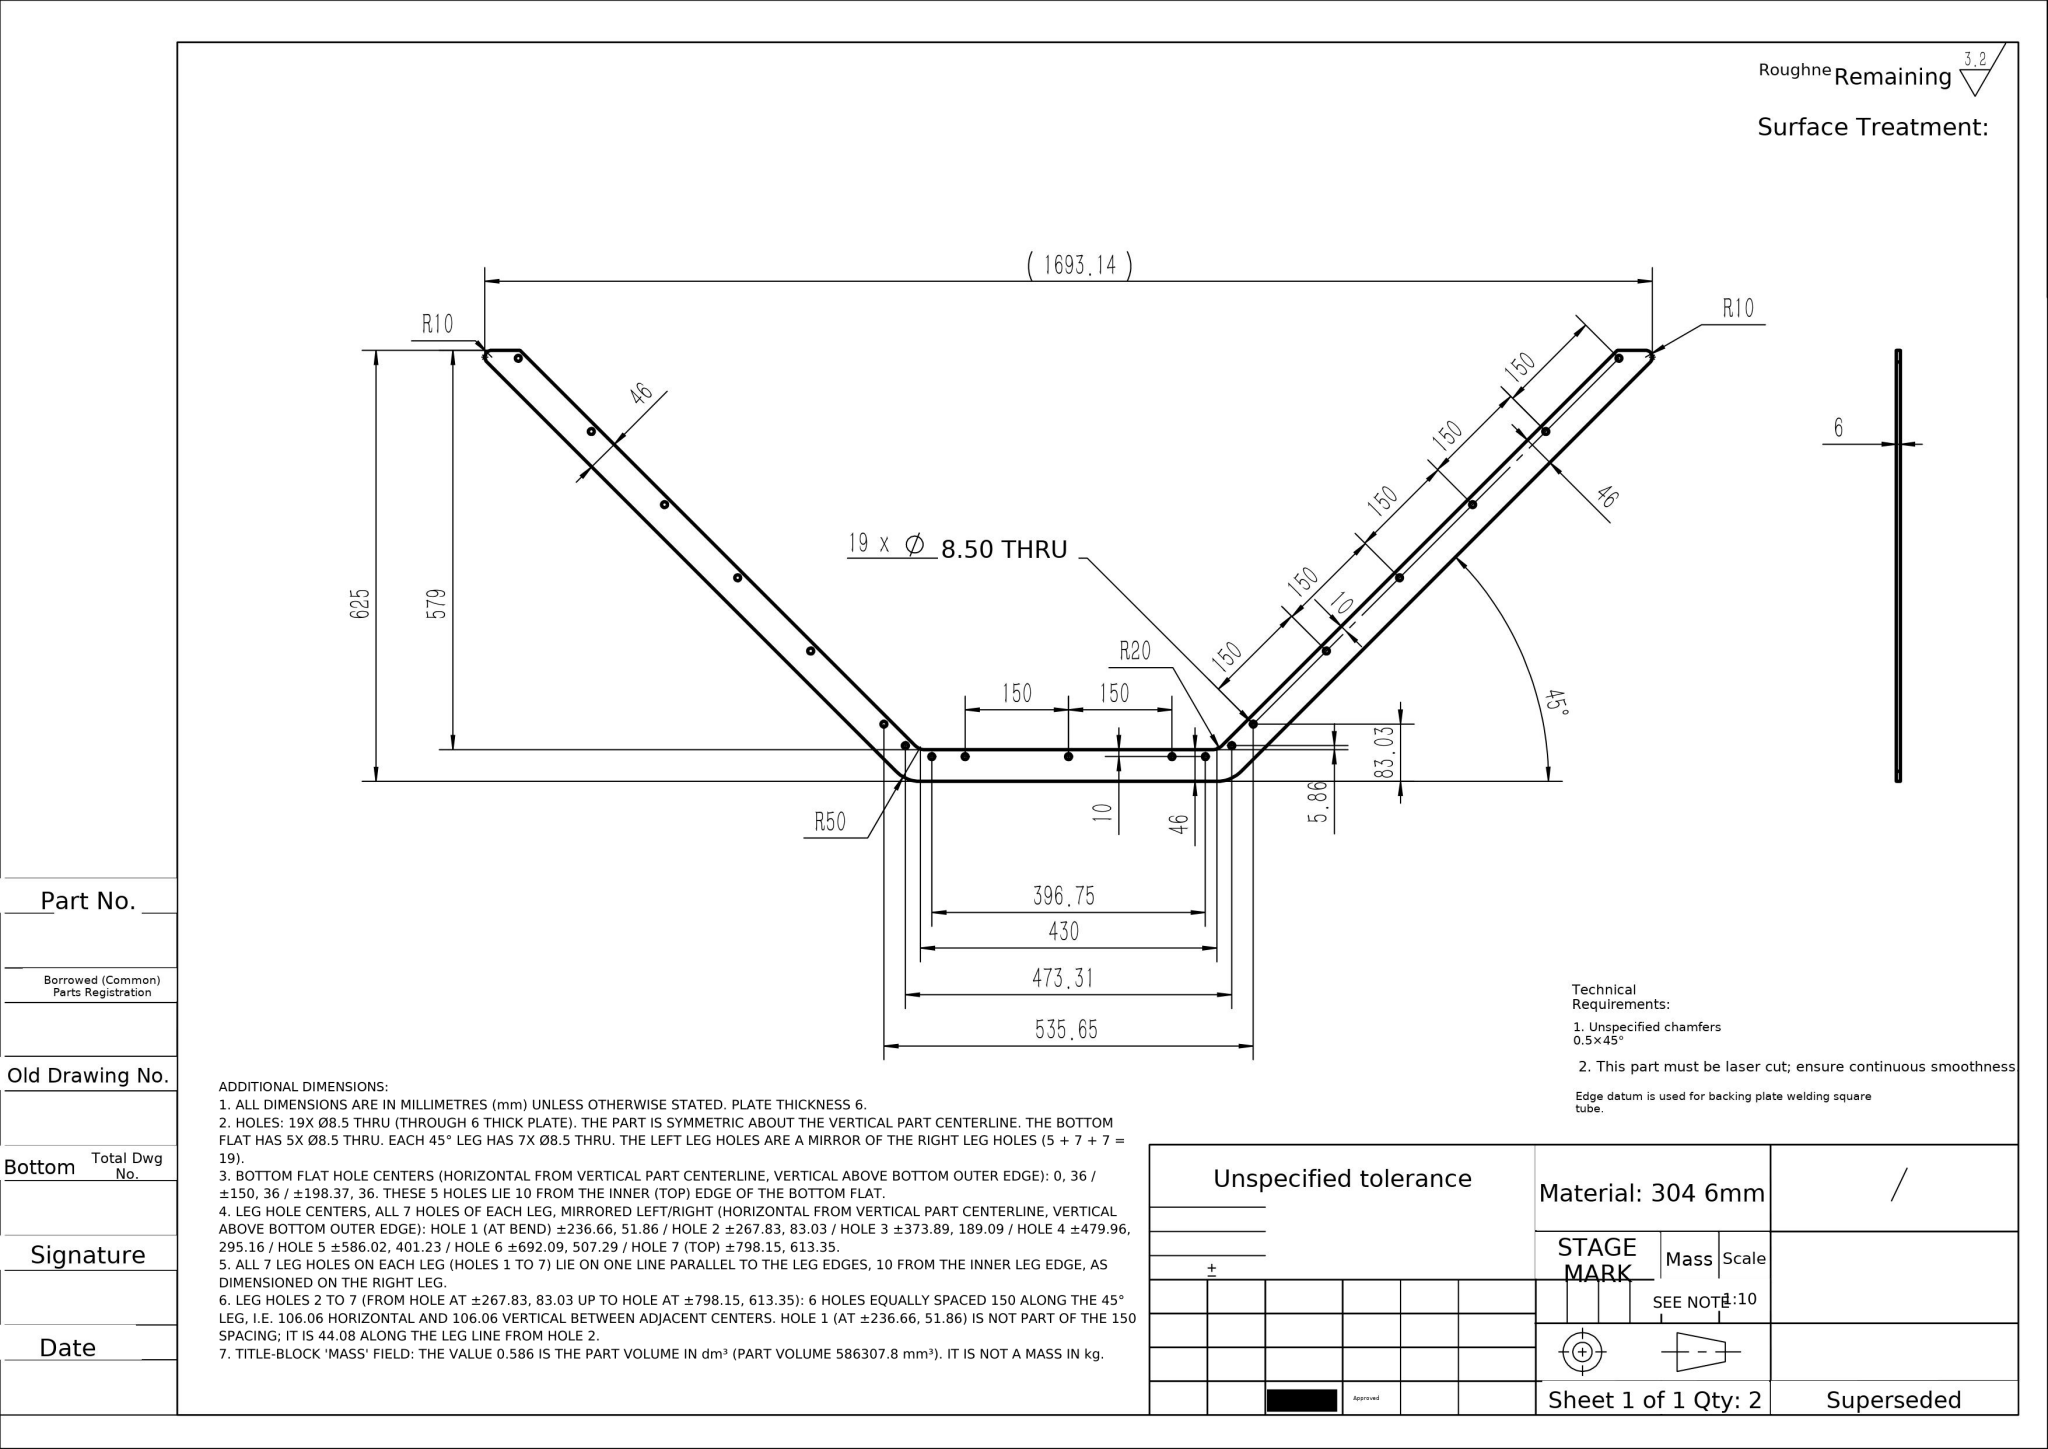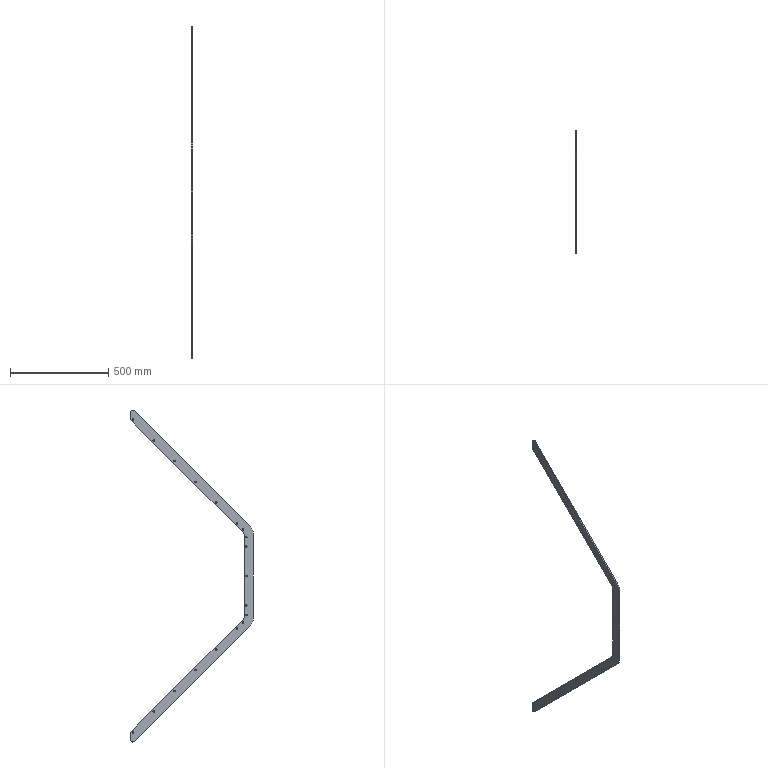Part | NX | mm | 1 solid | 55 faces | box 6 x 625 x 1693.14 mm | volume 586308 mm3 | cylinder 45 | plane 10 | commonest cylinder face diameters 8.5 x38 20 x3 100 x2 40 x2